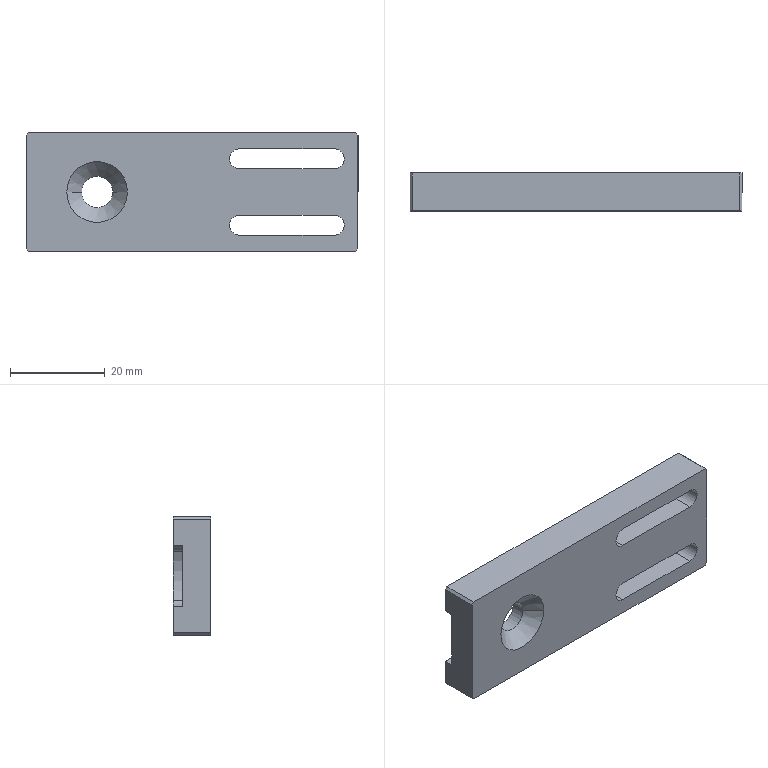Component | SolidWorks | QX1-24-TensionerSeat-1 | 1 solid | 30 faces | box 70 x 8 x 25 mm | volume 11297 mm3 | plane 17 | cylinder 11 | cone 2 | commonest cylinder face diameters 4.2 x6 6.6 x2 6 x2 19 x1 | material 6061 Alloy
build123d program:
from build123d import *

# Parameters (mm, degrees)
SKETCH1_W                                          = 70
SKETCH1_H                                          = 25
BOSS_EXTRUDE1_DEPTH                                = 8
CUT_EXTRUDE3_DEPTH                                 = 2
HOLE_SIZE_ACCORDING_TO_TYPE_1_OF_HEXAG_D           = 6.6
HOLE_SIZE_ACCORDING_TO_TYPE_1_OF_HEXAG_CSINK_D     = 12.8
HOLE_SIZE_ACCORDING_TO_TYPE_1_OF_HEXAG_CSINK_ANGLE = 90
FILLET1_R                                          = 3
CUT_EXTRUDE4_DEPTH                                 = 10
CHAMFER1_SIZE                                      = 0.5


with BuildPart() as part:
    # Sketch1 → Boss-Extrude1 (new body)
    with BuildSketch(Plane.XY):
        Rectangle(SKETCH1_W, SKETCH1_H)
    extrude(amount=BOSS_EXTRUDE1_DEPTH)

    # Sketch2 → Cut-Extrude3 (cut)
    with BuildSketch(Plane.XY.offset(8)):
        with BuildLine():
            Line((6.072, 6.5), (35, 6.5))
            Line((35, 6.5), (35, -6.5))
            Line((35, -6.5), (6.072, -6.5))
            ThreePointArc((6.072, -6.5), (3.5, 0), (6.072, 6.5))
        make_face()
    extrude(amount=-CUT_EXTRUDE3_DEPTH, mode=Mode.SUBTRACT)

    # Hole Size_ according to_ Type 1 of Hexag (through all)
    with Locations(Plane(origin=(0, 0, 0), x_dir=(-1, 0, 0), z_dir=(0, 0, -1))):
        with Locations((-20, 0)):
            CounterSinkHole(HOLE_SIZE_ACCORDING_TO_TYPE_1_OF_HEXAG_D / 2, HOLE_SIZE_ACCORDING_TO_TYPE_1_OF_HEXAG_CSINK_D / 2, counter_sink_angle=HOLE_SIZE_ACCORDING_TO_TYPE_1_OF_HEXAG_CSINK_ANGLE)

    # Fillet1
    fillet1_edges = [part.edges().sort_by_distance(p)[0] for p in [
        (6.072, -6.5, 7),
        (6.072, 6.5, 7),
    ]]
    fillet(fillet1_edges, radius=FILLET1_R)

    # Sketch7 → Cut-Extrude4 (cut)
    with BuildSketch(Plane.XY.offset(8)):
        with BuildLine():
            Line((-30, 9.1), (-10, 9.1))
            ThreePointArc((-10, 9.1), (-7.9, 7), (-10, 4.9))
            Line((-10, 4.9), (-30, 4.9))
            ThreePointArc((-30, 4.9), (-32.1, 7), (-30, 9.1))
        make_face()
    cut_extrude4 = extrude(amount=-CUT_EXTRUDE4_DEPTH, mode=Mode.SUBTRACT)

    # Mirror1: Cut-Extrude4 across plane
    add(cut_extrude4.mirror(Plane.ZX), mode=Mode.SUBTRACT)

    # Chamfer1
    chamfer1_edges = [part.edges().sort_by_distance(p)[0] for p in [
        (35, -12.5, 4),
        (-35, -12.5, 4),
        (-35, 12.5, 4),
        (35, 12.5, 4),
    ]]
    chamfer(chamfer1_edges, length=CHAMFER1_SIZE)


solid = part.part

# Placed as in the assembly
solid = solid.moved(Location((32.703, -35.916, 470.247), (-90, 0, 180)))
STEP:
#1=COLOUR_RGB('',0.7922,0.8196,0.9333);
#2=FILL_AREA_STYLE_COLOUR('',#1);
#3=FILL_AREA_STYLE('',(#2));
#4=SURFACE_STYLE_FILL_AREA(#3);
#5=SURFACE_SIDE_STYLE('',(#4));
#6=SURFACE_STYLE_USAGE(.BOTH.,#5);
#7=PRESENTATION_STYLE_ASSIGNMENT((#6));
#8=CARTESIAN_POINT('',(1.599,-1.414,18.238));
#9=VERTEX_POINT('',#8);
#10=CARTESIAN_POINT('',(1.681,-1.414,18.321));
#11=VERTEX_POINT('',#10);
#12=CARTESIAN_POINT('',(1.681,-1.414,18.238));
#13=DIRECTION('',(0.,1.,0.));
#14=DIRECTION('',(1.,0.,0.));
#15=AXIS2_PLACEMENT_3D('',#12,#13,#14);
#16=CIRCLE('',#15,0.08268);
#17=EDGE_CURVE('',#9,#11,#16,.T.);
#18=ORIENTED_EDGE('',*,*,#17,.F.);
#19=CARTESIAN_POINT('',(1.599,-1.099,18.238));
#20=VERTEX_POINT('',#19);
#21=CARTESIAN_POINT('',(1.599,-1.493,18.238));
#22=DIRECTION('',(0.,1.,0.));
#23=VECTOR('',#22,39.37);
#24=LINE('',#21,#23);
#25=EDGE_CURVE('',#9,#20,#24,.T.);
#26=ORIENTED_EDGE('',*,*,#25,.T.);
#27=CARTESIAN_POINT('',(1.681,-1.099,18.321));
#28=VERTEX_POINT('',#27);
#29=CARTESIAN_POINT('',(1.681,-1.099,18.238));
#30=DIRECTION('',(-0.,-1.,-0.));
#31=DIRECTION('',(-1.,0.,0.));
#32=AXIS2_PLACEMENT_3D('',#29,#30,#31);
#33=CIRCLE('',#32,0.08268);
#34=EDGE_CURVE('',#28,#20,#33,.T.);
#35=ORIENTED_EDGE('',*,*,#34,.F.);
#36=CARTESIAN_POINT('',(1.681,-1.493,18.321));
#37=DIRECTION('',(0.,1.,0.));
#38=VECTOR('',#37,39.37);
#39=LINE('',#36,#38);
#40=EDGE_CURVE('',#11,#28,#39,.T.);
#41=ORIENTED_EDGE('',*,*,#40,.F.);
#42=EDGE_LOOP('',(#18,#26,#35,#41));
#43=FACE_OUTER_BOUND('',#42,.T.);
#44=CARTESIAN_POINT('',(1.681,-1.493,18.238));
#45=DIRECTION('',(0.,1.,0.));
#46=DIRECTION('',(-1.,0.,0.));
#47=AXIS2_PLACEMENT_3D('',#44,#45,#46);
#48=CYLINDRICAL_SURFACE('',#47,0.08268);
#49=ADVANCED_FACE('',(#43),#48,.F.);
#50=CARTESIAN_POINT('',(1.681,-1.414,18.872));
#51=VERTEX_POINT('',#50);
#52=CARTESIAN_POINT('',(1.599,-1.414,18.789));
#53=VERTEX_POINT('',#52);
#54=CARTESIAN_POINT('',(1.681,-1.414,18.789));
#55=DIRECTION('',(-0.,-1.,-0.));
#56=DIRECTION('',(1.,0.,0.));
#57=AXIS2_PLACEMENT_3D('',#54,#55,#56);
#58=CIRCLE('',#57,0.08268);
#59=EDGE_CURVE('',#51,#53,#58,.T.);
#60=ORIENTED_EDGE('',*,*,#59,.T.);
#61=CARTESIAN_POINT('',(1.599,-1.099,18.789));
#62=VERTEX_POINT('',#61);
#63=CARTESIAN_POINT('',(1.599,-1.493,18.789));
#64=DIRECTION('',(0.,1.,0.));
#65=VECTOR('',#64,39.37);
#66=LINE('',#63,#65);
#67=EDGE_CURVE('',#53,#62,#66,.T.);
#68=ORIENTED_EDGE('',*,*,#67,.T.);
#69=CARTESIAN_POINT('',(1.681,-1.099,18.872));
#70=VERTEX_POINT('',#69);
#71=CARTESIAN_POINT('',(1.681,-1.099,18.789));
#72=DIRECTION('',(0.,1.,0.));
#73=DIRECTION('',(-1.,0.,0.));
#74=AXIS2_PLACEMENT_3D('',#71,#72,#73);
#75=CIRCLE('',#74,0.08268);
#76=EDGE_CURVE('',#62,#70,#75,.T.);
#77=ORIENTED_EDGE('',*,*,#76,.T.);
#78=CARTESIAN_POINT('',(1.681,-1.493,18.872));
#79=DIRECTION('',(0.,1.,0.));
#80=VECTOR('',#79,39.37);
#81=LINE('',#78,#80);
#82=EDGE_CURVE('',#51,#70,#81,.T.);
#83=ORIENTED_EDGE('',*,*,#82,.F.);
#84=EDGE_LOOP('',(#60,#68,#77,#83));
#85=FACE_OUTER_BOUND('',#84,.T.);
#86=CARTESIAN_POINT('',(1.681,-1.493,18.789));
#87=DIRECTION('',(0.,1.,0.));
#88=DIRECTION('',(-1.,0.,0.));
#89=AXIS2_PLACEMENT_3D('',#86,#87,#88);
#90=CYLINDRICAL_SURFACE('',#89,0.08268);
#91=ADVANCED_FACE('',(#85),#90,.F.);
#92=CARTESIAN_POINT('',(0.3702,-1.292,18.514));
#93=VERTEX_POINT('',#92);
#94=CARTESIAN_POINT('',(0.6301,-1.292,18.514));
#95=VERTEX_POINT('',#94);
#96=CARTESIAN_POINT('',(0.5001,-1.292,18.514));
#97=DIRECTION('',(-0.,-1.,-0.));
#98=DIRECTION('',(1.,0.,0.));
#99=AXIS2_PLACEMENT_3D('',#96,#97,#98);
#100=CIRCLE('',#99,0.1299);
#101=EDGE_CURVE('',#93,#95,#100,.T.);
#102=ORIENTED_EDGE('',*,*,#101,.F.);
#103=CARTESIAN_POINT('',(0.2482,-1.414,18.514));
#104=VERTEX_POINT('',#103);
#105=CARTESIAN_POINT('',(0.2482,-1.414,18.514));
#106=DIRECTION('',(-0.7071,-0.7071,0.));
#107=VECTOR('',#106,39.37);
#108=LINE('',#105,#107);
#109=EDGE_CURVE('',#93,#104,#108,.T.);
#110=ORIENTED_EDGE('',*,*,#109,.T.);
#111=CARTESIAN_POINT('',(0.7521,-1.414,18.514));
#112=VERTEX_POINT('',#111);
#113=CARTESIAN_POINT('',(0.5001,-1.414,18.514));
#114=DIRECTION('',(-0.,-1.,-0.));
#115=DIRECTION('',(1.,-0.,0.));
#116=AXIS2_PLACEMENT_3D('',#113,#114,#115);
#117=CIRCLE('',#116,0.252);
#118=EDGE_CURVE('',#104,#112,#117,.T.);
#119=ORIENTED_EDGE('',*,*,#118,.T.);
#120=CARTESIAN_POINT('',(0.7521,-1.414,18.514));
#121=DIRECTION('',(0.7071,-0.7071,-0.));
#122=VECTOR('',#121,39.37);
#123=LINE('',#120,#122);
#124=EDGE_CURVE('',#95,#112,#123,.T.);
#125=ORIENTED_EDGE('',*,*,#124,.F.);
#126=EDGE_LOOP('',(#102,#110,#119,#125));
#127=FACE_OUTER_BOUND('',#126,.T.);
#128=CARTESIAN_POINT('',(0.5001,-1.414,18.514));
#129=DIRECTION('',(-0.,-1.,-0.));
#130=DIRECTION('',(1.,-0.,0.));
#131=AXIS2_PLACEMENT_3D('',#128,#129,#130);
#132=CONICAL_SURFACE('',#131,0.252,0.7854);
#133=ADVANCED_FACE('',(#127),#132,.F.);
#134=CARTESIAN_POINT('',(0.6301,-1.178,18.514));
#135=VERTEX_POINT('',#134);
#136=CARTESIAN_POINT('',(0.3702,-1.178,18.514));
#137=VERTEX_POINT('',#136);
#138=CARTESIAN_POINT('',(0.5001,-1.178,18.514));
#139=DIRECTION('',(0.,1.,0.));
#140=DIRECTION('',(-1.,0.,0.));
#141=AXIS2_PLACEMENT_3D('',#138,#139,#140);
#142=CIRCLE('',#141,0.1299);
#143=EDGE_CURVE('',#135,#137,#142,.T.);
#144=ORIENTED_EDGE('',*,*,#143,.T.);
#145=CARTESIAN_POINT('',(0.3702,-1.414,18.514));
#146=DIRECTION('',(-0.,-1.,-0.));
#147=VECTOR('',#146,39.37);
#148=LINE('',#145,#147);
#149=EDGE_CURVE('',#137,#93,#148,.T.);
#150=ORIENTED_EDGE('',*,*,#149,.T.);
#151=ORIENTED_EDGE('',*,*,#101,.T.);
#152=CARTESIAN_POINT('',(0.6301,-1.414,18.514));
#153=DIRECTION('',(-0.,-1.,-0.));
#154=VECTOR('',#153,39.37);
#155=LINE('',#152,#154);
#156=EDGE_CURVE('',#135,#95,#155,.T.);
#157=ORIENTED_EDGE('',*,*,#156,.F.);
#158=EDGE_LOOP('',(#144,#150,#151,#157));
#159=FACE_OUTER_BOUND('',#158,.T.);
#160=CARTESIAN_POINT('',(0.5001,-1.414,18.514));
#161=DIRECTION('',(-0.,-1.,-0.));
#162=DIRECTION('',(1.,0.,0.));
#163=AXIS2_PLACEMENT_3D('',#160,#161,#162);
#164=CYLINDRICAL_SURFACE('',#163,0.1299);
#165=ADVANCED_FACE('',(#159),#164,.F.);
#166=CARTESIAN_POINT('',(-0.09042,-1.099,18.77));
#167=VERTEX_POINT('',#166);
#168=CARTESIAN_POINT('',(-0.09042,-1.099,18.986));
#169=VERTEX_POINT('',#168);
#170=CARTESIAN_POINT('',(-0.09042,-1.099,18.022));
#171=DIRECTION('',(0.,-0.,1.));
#172=VECTOR('',#171,39.37);
#173=LINE('',#170,#172);
#174=EDGE_CURVE('',#167,#169,#173,.T.);
#175=ORIENTED_EDGE('',*,*,#174,.T.);
#176=CARTESIAN_POINT('',(-0.07074,-1.099,19.006));
#177=VERTEX_POINT('',#176);
#178=CARTESIAN_POINT('',(-0.07074,-1.099,19.006));
#179=DIRECTION('',(0.7071,-0.,0.7071));
#180=VECTOR('',#179,39.37);
#181=LINE('',#178,#180);
#182=EDGE_CURVE('',#169,#177,#181,.T.);
#183=ORIENTED_EDGE('',*,*,#182,.T.);
#184=CARTESIAN_POINT('',(2.646,-1.099,19.006));
#185=VERTEX_POINT('',#184);
#186=CARTESIAN_POINT('',(2.665,-1.099,19.006));
#187=DIRECTION('',(1.,-0.,-0.));
#188=VECTOR('',#187,39.37);
#189=LINE('',#186,#188);
#190=EDGE_CURVE('',#177,#185,#189,.T.);
#191=ORIENTED_EDGE('',*,*,#190,.T.);
#192=CARTESIAN_POINT('',(2.665,-1.099,18.986));
#193=VERTEX_POINT('',#192);
#194=CARTESIAN_POINT('',(2.665,-1.099,18.986));
#195=DIRECTION('',(0.7071,-0.,-0.7071));
#196=VECTOR('',#195,39.37);
#197=LINE('',#194,#196);
#198=EDGE_CURVE('',#185,#193,#197,.T.);
#199=ORIENTED_EDGE('',*,*,#198,.T.);
#200=CARTESIAN_POINT('',(2.665,-1.099,18.041));
#201=VERTEX_POINT('',#200);
#202=CARTESIAN_POINT('',(2.665,-1.099,18.022));
#203=DIRECTION('',(-0.,0.,-1.));
#204=VECTOR('',#203,39.37);
#205=LINE('',#202,#204);
#206=EDGE_CURVE('',#193,#201,#205,.T.);
#207=ORIENTED_EDGE('',*,*,#206,.T.);
#208=CARTESIAN_POINT('',(2.646,-1.099,18.022));
#209=VERTEX_POINT('',#208);
#210=CARTESIAN_POINT('',(2.646,-1.099,18.022));
#211=DIRECTION('',(-0.7071,0.,-0.7071));
#212=VECTOR('',#211,39.37);
#213=LINE('',#210,#212);
#214=EDGE_CURVE('',#201,#209,#213,.T.);
#215=ORIENTED_EDGE('',*,*,#214,.T.);
#216=CARTESIAN_POINT('',(-0.07074,-1.099,18.022));
#217=VERTEX_POINT('',#216);
#218=CARTESIAN_POINT('',(2.665,-1.099,18.022));
#219=DIRECTION('',(-1.,0.,0.));
#220=VECTOR('',#219,39.37);
#221=LINE('',#218,#220);
#222=EDGE_CURVE('',#209,#217,#221,.T.);
#223=ORIENTED_EDGE('',*,*,#222,.T.);
#224=CARTESIAN_POINT('',(-0.09042,-1.099,18.041));
#225=VERTEX_POINT('',#224);
#226=CARTESIAN_POINT('',(-0.09042,-1.099,18.041));
#227=DIRECTION('',(-0.7071,0.,0.7071));
#228=VECTOR('',#227,39.37);
#229=LINE('',#226,#228);
#230=EDGE_CURVE('',#217,#225,#229,.T.);
#231=ORIENTED_EDGE('',*,*,#230,.T.);
#232=CARTESIAN_POINT('',(-0.09042,-1.099,18.258));
#233=VERTEX_POINT('',#232);
#234=CARTESIAN_POINT('',(-0.09042,-1.099,18.022));
#235=DIRECTION('',(0.,-0.,1.));
#236=VECTOR('',#235,39.37);
#237=LINE('',#234,#236);
#238=EDGE_CURVE('',#225,#233,#237,.T.);
#239=ORIENTED_EDGE('',*,*,#238,.T.);
#240=CARTESIAN_POINT('',(0.9914,-1.099,18.258));
#241=VERTEX_POINT('',#240);
#242=CARTESIAN_POINT('',(1.048,-1.099,18.258));
#243=DIRECTION('',(-1.,0.,0.));
#244=VECTOR('',#243,39.37);
#245=LINE('',#242,#244);
#246=EDGE_CURVE('',#241,#233,#245,.T.);
#247=ORIENTED_EDGE('',*,*,#246,.F.);
#248=CARTESIAN_POINT('',(1.091,-1.099,18.312));
#249=VERTEX_POINT('',#248);
#250=CARTESIAN_POINT('',(0.9914,-1.099,18.376));
#251=DIRECTION('',(-0.,-1.,-0.));
#252=DIRECTION('',(1.,-0.,0.));
#253=AXIS2_PLACEMENT_3D('',#250,#251,#252);
#254=CIRCLE('',#253,0.1181);
#255=EDGE_CURVE('',#241,#249,#254,.T.);
#256=ORIENTED_EDGE('',*,*,#255,.T.);
#257=CARTESIAN_POINT('',(1.091,-1.099,18.715));
#258=VERTEX_POINT('',#257);
#259=CARTESIAN_POINT('',(0.7757,-1.099,18.514));
#260=DIRECTION('',(0.,1.,0.));
#261=DIRECTION('',(-1.,0.,0.));
#262=AXIS2_PLACEMENT_3D('',#259,#260,#261);
#263=CIRCLE('',#262,0.374);
#264=EDGE_CURVE('',#258,#249,#263,.T.);
#265=ORIENTED_EDGE('',*,*,#264,.F.);
#266=CARTESIAN_POINT('',(0.9914,-1.099,18.77));
#267=VERTEX_POINT('',#266);
#268=CARTESIAN_POINT('',(0.9914,-1.099,18.651));
#269=DIRECTION('',(-0.,-1.,-0.));
#270=DIRECTION('',(1.,-0.,0.));
#271=AXIS2_PLACEMENT_3D('',#268,#269,#270);
#272=CIRCLE('',#271,0.1181);
#273=EDGE_CURVE('',#258,#267,#272,.T.);
#274=ORIENTED_EDGE('',*,*,#273,.T.);
#275=CARTESIAN_POINT('',(1.048,-1.099,18.77));
#276=DIRECTION('',(-1.,0.,0.));
#277=VECTOR('',#276,39.37);
#278=LINE('',#275,#277);
#279=EDGE_CURVE('',#267,#167,#278,.T.);
#280=ORIENTED_EDGE('',*,*,#279,.T.);
#281=EDGE_LOOP('',(#175,#183,#191,#199,#207,#215,#223,#231,#239,#247,#256,#265,#274,#280));
#282=FACE_OUTER_BOUND('',#281,.T.);
#283=CARTESIAN_POINT('',(2.469,-1.099,18.707));
#284=VERTEX_POINT('',#283);
#285=CARTESIAN_POINT('',(1.681,-1.099,18.707));
#286=VERTEX_POINT('',#285);
#287=CARTESIAN_POINT('',(2.469,-1.099,18.707));
#288=DIRECTION('',(-1.,0.,0.));
#289=VECTOR('',#288,39.37);
#290=LINE('',#287,#289);
#291=EDGE_CURVE('',#284,#286,#290,.T.);
#292=ORIENTED_EDGE('',*,*,#291,.F.);
#293=CARTESIAN_POINT('',(2.469,-1.099,18.872));
#294=VERTEX_POINT('',#293);
#295=CARTESIAN_POINT('',(2.469,-1.099,18.789));
#296=DIRECTION('',(0.,1.,0.));
#297=DIRECTION('',(-1.,0.,0.));
#298=AXIS2_PLACEMENT_3D('',#295,#296,#297);
#299=CIRCLE('',#298,0.08268);
#300=EDGE_CURVE('',#294,#284,#299,.T.);
#301=ORIENTED_EDGE('',*,*,#300,.F.);
#302=CARTESIAN_POINT('',(2.469,-1.099,18.872));
#303=DIRECTION('',(1.,-0.,-0.));
#304=VECTOR('',#303,39.37);
#305=LINE('',#302,#304);
#306=EDGE_CURVE('',#70,#294,#305,.T.);
#307=ORIENTED_EDGE('',*,*,#306,.F.);
#308=ORIENTED_EDGE('',*,*,#76,.F.);
#309=CARTESIAN_POINT('',(1.681,-1.099,18.789));
#310=DIRECTION('',(0.,1.,0.));
#311=DIRECTION('',(-1.,0.,0.));
#312=AXIS2_PLACEMENT_3D('',#309,#310,#311);
#313=CIRCLE('',#312,0.08268);
#314=EDGE_CURVE('',#286,#62,#313,.T.);
#315=ORIENTED_EDGE('',*,*,#314,.F.);
#316=EDGE_LOOP('',(#292,#301,#307,#308,#315));
#317=FACE_BOUND('',#316,.T.);
#318=CARTESIAN_POINT('',(2.469,-1.099,18.155));
#319=VERTEX_POINT('',#318);
#320=CARTESIAN_POINT('',(2.469,-1.099,18.321));
#321=VERTEX_POINT('',#320);
#322=CARTESIAN_POINT('',(2.469,-1.099,18.238));
#323=DIRECTION('',(-0.,-1.,-0.));
#324=DIRECTION('',(-1.,0.,0.));
#325=AXIS2_PLACEMENT_3D('',#322,#323,#324);
#326=CIRCLE('',#325,0.08268);
#327=EDGE_CURVE('',#319,#321,#326,.T.);
#328=ORIENTED_EDGE('',*,*,#327,.T.);
#329=CARTESIAN_POINT('',(2.469,-1.099,18.321));
#330=DIRECTION('',(-1.,0.,0.));
#331=VECTOR('',#330,39.37);
#332=LINE('',#329,#331);
#333=EDGE_CURVE('',#321,#28,#332,.T.);
#334=ORIENTED_EDGE('',*,*,#333,.T.);
#335=ORIENTED_EDGE('',*,*,#34,.T.);
#336=CARTESIAN_POINT('',(1.681,-1.099,18.155));
#337=VERTEX_POINT('',#336);
#338=CARTESIAN_POINT('',(1.681,-1.099,18.238));
#339=DIRECTION('',(-0.,-1.,-0.));
#340=DIRECTION('',(-1.,0.,0.));
#341=AXIS2_PLACEMENT_3D('',#338,#339,#340);
#342=CIRCLE('',#341,0.08268);
#343=EDGE_CURVE('',#20,#337,#342,.T.);
#344=ORIENTED_EDGE('',*,*,#343,.T.);
#345=CARTESIAN_POINT('',(2.469,-1.099,18.155));
#346=DIRECTION('',(1.,-0.,-0.));
#347=VECTOR('',#346,39.37);
#348=LINE('',#345,#347);
#349=EDGE_CURVE('',#337,#319,#348,.T.);
#350=ORIENTED_EDGE('',*,*,#349,.T.);
#351=EDGE_LOOP('',(#328,#334,#335,#344,#350));
#352=FACE_BOUND('',#351,.T.);
#353=CARTESIAN_POINT('',(1.288,-1.099,18.514));
#354=DIRECTION('',(-0.,-1.,-0.));
#355=DIRECTION('',(1.,-0.,-0.));
#356=AXIS2_PLACEMENT_3D('',#353,#354,#355);
#357=PLANE('',#356);
#358=ADVANCED_FACE('',(#282,#317,#352),#357,.F.);
#359=CARTESIAN_POINT('',(2.469,-1.414,18.707));
#360=VERTEX_POINT('',#359);
#361=CARTESIAN_POINT('',(2.469,-1.414,18.872));
#362=VERTEX_POINT('',#361);
#363=CARTESIAN_POINT('',(2.469,-1.414,18.789));
#364=DIRECTION('',(-0.,-1.,-0.));
#365=DIRECTION('',(1.,0.,0.));
#366=AXIS2_PLACEMENT_3D('',#363,#364,#365);
#367=CIRCLE('',#366,0.08268);
#368=EDGE_CURVE('',#360,#362,#367,.T.);
#369=ORIENTED_EDGE('',*,*,#368,.F.);
#370=CARTESIAN_POINT('',(1.681,-1.414,18.707));
#371=VERTEX_POINT('',#370);
#372=CARTESIAN_POINT('',(1.288,-1.414,18.707));
#373=DIRECTION('',(1.,-0.,-0.));
#374=VECTOR('',#373,39.37);
#375=LINE('',#372,#374);
#376=EDGE_CURVE('',#371,#360,#375,.T.);
#377=ORIENTED_EDGE('',*,*,#376,.F.);
#378=CARTESIAN_POINT('',(1.681,-1.414,18.789));
#379=DIRECTION('',(-0.,-1.,-0.));
#380=DIRECTION('',(1.,0.,0.));
#381=AXIS2_PLACEMENT_3D('',#378,#379,#380);
#382=CIRCLE('',#381,0.08268);
#383=EDGE_CURVE('',#53,#371,#382,.T.);
#384=ORIENTED_EDGE('',*,*,#383,.F.);
#385=ORIENTED_EDGE('',*,*,#59,.F.);
#386=CARTESIAN_POINT('',(1.288,-1.414,18.872));
#387=DIRECTION('',(-1.,0.,0.));
#388=VECTOR('',#387,39.37);
#389=LINE('',#386,#388);
#390=EDGE_CURVE('',#362,#51,#389,.T.);
#391=ORIENTED_EDGE('',*,*,#390,.F.);
#392=EDGE_LOOP('',(#369,#377,#384,#385,#391));
#393=FACE_BOUND('',#392,.T.);
#394=CARTESIAN_POINT('',(0.5001,-1.414,18.514));
#395=DIRECTION('',(-0.,-1.,-0.));
#396=DIRECTION('',(1.,-0.,0.));
#397=AXIS2_PLACEMENT_3D('',#394,#395,#396);
#398=CIRCLE('',#397,0.252);
#399=EDGE_CURVE('',#112,#104,#398,.T.);
#400=ORIENTED_EDGE('',*,*,#399,.F.);
#401=ORIENTED_EDGE('',*,*,#118,.F.);
#402=EDGE_LOOP('',(#400,#401));
#403=FACE_BOUND('',#402,.T.);
#404=CARTESIAN_POINT('',(-0.07074,-1.414,19.006));
#405=VERTEX_POINT('',#404);
#406=CARTESIAN_POINT('',(2.646,-1.414,19.006));
#407=VERTEX_POINT('',#406);
#408=CARTESIAN_POINT('',(2.665,-1.414,19.006));
#409=DIRECTION('',(1.,-0.,-0.));
#410=VECTOR('',#409,39.37);
#411=LINE('',#408,#410);
#412=EDGE_CURVE('',#405,#407,#411,.T.);
#413=ORIENTED_EDGE('',*,*,#412,.F.);
#414=CARTESIAN_POINT('',(-0.09042,-1.414,18.986));
#415=VERTEX_POINT('',#414);
#416=CARTESIAN_POINT('',(0.3623,-1.414,19.439));
#417=DIRECTION('',(-0.7071,0.,-0.7071));
#418=VECTOR('',#417,39.37);
#419=LINE('',#416,#418);
#420=EDGE_CURVE('',#405,#415,#419,.T.);
#421=ORIENTED_EDGE('',*,*,#420,.T.);
#422=CARTESIAN_POINT('',(-0.09042,-1.414,18.041));
#423=VERTEX_POINT('',#422);
#424=CARTESIAN_POINT('',(-0.09042,-1.414,18.022));
#425=DIRECTION('',(0.,-0.,1.));
#426=VECTOR('',#425,39.37);
#427=LINE('',#424,#426);
#428=EDGE_CURVE('',#423,#415,#427,.T.);
#429=ORIENTED_EDGE('',*,*,#428,.F.);
#430=CARTESIAN_POINT('',(-0.07074,-1.414,18.022));
#431=VERTEX_POINT('',#430);
#432=CARTESIAN_POINT('',(0.3623,-1.414,17.588));
#433=DIRECTION('',(0.7071,-0.,-0.7071));
#434=VECTOR('',#433,39.37);
#435=LINE('',#432,#434);
#436=EDGE_CURVE('',#423,#431,#435,.T.);
#437=ORIENTED_EDGE('',*,*,#436,.T.);
#438=CARTESIAN_POINT('',(2.646,-1.414,18.022));
#439=VERTEX_POINT('',#438);
#440=CARTESIAN_POINT('',(2.665,-1.414,18.022));
#441=DIRECTION('',(-1.,0.,0.));
#442=VECTOR('',#441,39.37);
#443=LINE('',#440,#442);
#444=EDGE_CURVE('',#439,#431,#443,.T.);
#445=ORIENTED_EDGE('',*,*,#444,.F.);
#446=CARTESIAN_POINT('',(2.665,-1.414,18.041));
#447=VERTEX_POINT('',#446);
#448=CARTESIAN_POINT('',(2.213,-1.414,17.588));
#449=DIRECTION('',(0.7071,-0.,0.7071));
#450=VECTOR('',#449,39.37);
#451=LINE('',#448,#450);
#452=EDGE_CURVE('',#439,#447,#451,.T.);
#453=ORIENTED_EDGE('',*,*,#452,.T.);
#454=CARTESIAN_POINT('',(2.665,-1.414,18.986));
#455=VERTEX_POINT('',#454);
#456=CARTESIAN_POINT('',(2.665,-1.414,18.022));
#457=DIRECTION('',(-0.,0.,-1.));
#458=VECTOR('',#457,39.37);
#459=LINE('',#456,#458);
#460=EDGE_CURVE('',#455,#447,#459,.T.);
#461=ORIENTED_EDGE('',*,*,#460,.F.);
#462=CARTESIAN_POINT('',(2.213,-1.414,19.439));
#463=DIRECTION('',(-0.7071,0.,0.7071));
#464=VECTOR('',#463,39.37);
#465=LINE('',#462,#464);
#466=EDGE_CURVE('',#455,#407,#465,.T.);
#467=ORIENTED_EDGE('',*,*,#466,.T.);
#468=EDGE_LOOP('',(#413,#421,#429,#437,#445,#453,#461,#467));
#469=FACE_OUTER_BOUND('',#468,.T.);
#470=CARTESIAN_POINT('',(2.469,-1.414,18.321));
#471=VERTEX_POINT('',#470);
#472=CARTESIAN_POINT('',(1.288,-1.414,18.321));
#473=DIRECTION('',(1.,-0.,-0.));
#474=VECTOR('',#473,39.37);
#475=LINE('',#472,#474);
#476=EDGE_CURVE('',#11,#471,#475,.T.);
#477=ORIENTED_EDGE('',*,*,#476,.T.);
#478=CARTESIAN_POINT('',(2.469,-1.414,18.155));
#479=VERTEX_POINT('',#478);
#480=CARTESIAN_POINT('',(2.469,-1.414,18.238));
#481=DIRECTION('',(0.,1.,0.));
#482=DIRECTION('',(1.,0.,0.));
#483=AXIS2_PLACEMENT_3D('',#480,#481,#482);
#484=CIRCLE('',#483,0.08268);
#485=EDGE_CURVE('',#471,#479,#484,.T.);
#486=ORIENTED_EDGE('',*,*,#485,.T.);
#487=CARTESIAN_POINT('',(1.681,-1.414,18.155));
#488=VERTEX_POINT('',#487);
#489=CARTESIAN_POINT('',(1.288,-1.414,18.155));
#490=DIRECTION('',(-1.,0.,0.));
#491=VECTOR('',#490,39.37);
#492=LINE('',#489,#491);
#493=EDGE_CURVE('',#479,#488,#492,.T.);
#494=ORIENTED_EDGE('',*,*,#493,.T.);
#495=CARTESIAN_POINT('',(1.681,-1.414,18.238));
#496=DIRECTION('',(0.,1.,0.));
#497=DIRECTION('',(1.,0.,0.));
#498=AXIS2_PLACEMENT_3D('',#495,#496,#497);
#499=CIRCLE('',#498,0.08268);
#500=EDGE_CURVE('',#488,#9,#499,.T.);
#501=ORIENTED_EDGE('',*,*,#500,.T.);
#502=ORIENTED_EDGE('',*,*,#17,.T.);
#503=EDGE_LOOP('',(#477,#486,#494,#501,#502));
#504=FACE_BOUND('',#503,.T.);
#505=CARTESIAN_POINT('',(1.288,-1.414,18.514));
#506=DIRECTION('',(-0.,-1.,-0.));
#507=DIRECTION('',(1.,-0.,-0.));
#508=AXIS2_PLACEMENT_3D('',#505,#506,#507);
#509=PLANE('',#508);
#510=ADVANCED_FACE('',(#393,#403,#469,#504),#509,.T.);
#511=ORIENTED_EDGE('',*,*,#428,.T.);
#512=CARTESIAN_POINT('',(-0.09042,-1.099,18.986));
#513=DIRECTION('',(0.,1.,0.));
#514=VECTOR('',#513,39.37);
#515=LINE('',#512,#514);
#516=EDGE_CURVE('',#415,#169,#515,.T.);
#517=ORIENTED_EDGE('',*,*,#516,.T.);
#518=ORIENTED_EDGE('',*,*,#174,.F.);
#519=CARTESIAN_POINT('',(-0.09042,-1.178,18.77));
#520=VERTEX_POINT('',#519);
#521=CARTESIAN_POINT('',(-0.09042,-1.178,18.77));
#522=DIRECTION('',(0.,1.,0.));
#523=VECTOR('',#522,39.37);
#524=LINE('',#521,#523);
#525=EDGE_CURVE('',#520,#167,#524,.T.);
#526=ORIENTED_EDGE('',*,*,#525,.F.);
#527=CARTESIAN_POINT('',(-0.09042,-1.178,18.258));
#528=VERTEX_POINT('',#527);
#529=CARTESIAN_POINT('',(-0.09042,-1.178,18.77));
#530=DIRECTION('',(-0.,0.,-1.));
#531=VECTOR('',#530,39.37);
#532=LINE('',#529,#531);
#533=EDGE_CURVE('',#520,#528,#532,.T.);
#534=ORIENTED_EDGE('',*,*,#533,.T.);
#535=CARTESIAN_POINT('',(-0.09042,-1.178,18.258));
#536=DIRECTION('',(0.,1.,0.));
#537=VECTOR('',#536,39.37);
#538=LINE('',#535,#537);
#539=EDGE_CURVE('',#528,#233,#538,.T.);
#540=ORIENTED_EDGE('',*,*,#539,.T.);
#541=ORIENTED_EDGE('',*,*,#238,.F.);
#542=CARTESIAN_POINT('',(-0.09042,-1.099,18.041));
#543=DIRECTION('',(-0.,-1.,-0.));
#544=VECTOR('',#543,39.37);
#545=LINE('',#542,#544);
#546=EDGE_CURVE('',#225,#423,#545,.T.);
#547=ORIENTED_EDGE('',*,*,#546,.T.);
#548=EDGE_LOOP('',(#511,#517,#518,#526,#534,#540,#541,#547));
#549=FACE_OUTER_BOUND('',#548,.T.);
#550=CARTESIAN_POINT('',(-0.09042,-1.099,18.022));
#551=DIRECTION('',(1.,-0.,-0.));
#552=DIRECTION('',(0.,1.,0.));
#553=AXIS2_PLACEMENT_3D('',#550,#551,#552);
#554=PLANE('',#553);
#555=ADVANCED_FACE('',(#549),#554,.F.);
#556=ORIENTED_EDGE('',*,*,#190,.F.);
#557=CARTESIAN_POINT('',(-0.07074,-1.099,19.006));
#558=DIRECTION('',(-0.,-1.,-0.));
#559=VECTOR('',#558,39.37);
#560=LINE('',#557,#559);
#561=EDGE_CURVE('',#177,#405,#560,.T.);
#562=ORIENTED_EDGE('',*,*,#561,.T.);
#563=ORIENTED_EDGE('',*,*,#412,.T.);
#564=CARTESIAN_POINT('',(2.646,-1.099,19.006));
#565=DIRECTION('',(0.,1.,0.));
#566=VECTOR('',#565,39.37);
#567=LINE('',#564,#566);
#568=EDGE_CURVE('',#407,#185,#567,.T.);
#569=ORIENTED_EDGE('',*,*,#568,.T.);
#570=EDGE_LOOP('',(#556,#562,#563,#569));
#571=FACE_OUTER_BOUND('',#570,.T.);
#572=CARTESIAN_POINT('',(2.665,-1.099,19.006));
#573=DIRECTION('',(-0.,0.,-1.));
#574=DIRECTION('',(-0.,-1.,-0.));
#575=AXIS2_PLACEMENT_3D('',#572,#573,#574);
#576=PLANE('',#575);
#577=ADVANCED_FACE('',(#571),#576,.F.);
#578=ORIENTED_EDGE('',*,*,#460,.T.);
#579=CARTESIAN_POINT('',(2.665,-1.099,18.041));
#580=DIRECTION('',(0.,1.,0.));
#581=VECTOR('',#580,39.37);
#582=LINE('',#579,#581);
#583=EDGE_CURVE('',#447,#201,#582,.T.);
#584=ORIENTED_EDGE('',*,*,#583,.T.);
#585=ORIENTED_EDGE('',*,*,#206,.F.);
#586=CARTESIAN_POINT('',(2.665,-1.099,18.986));
#587=DIRECTION('',(-0.,-1.,-0.));
#588=VECTOR('',#587,39.37);
#589=LINE('',#586,#588);
#590=EDGE_CURVE('',#193,#455,#589,.T.);
#591=ORIENTED_EDGE('',*,*,#590,.T.);
#592=EDGE_LOOP('',(#578,#584,#585,#591));
#593=FACE_OUTER_BOUND('',#592,.T.);
#594=CARTESIAN_POINT('',(2.665,-1.099,18.022));
#595=DIRECTION('',(-1.,0.,0.));
#596=DIRECTION('',(-0.,-1.,-0.));
#597=AXIS2_PLACEMENT_3D('',#594,#595,#596);
#598=PLANE('',#597);
#599=ADVANCED_FACE('',(#593),#598,.F.);
#600=ORIENTED_EDGE('',*,*,#444,.T.);
#601=CARTESIAN_POINT('',(-0.07074,-1.099,18.022));
#602=DIRECTION('',(0.,1.,0.));
#603=VECTOR('',#602,39.37);
#604=LINE('',#601,#603);
#605=EDGE_CURVE('',#431,#217,#604,.T.);
#606=ORIENTED_EDGE('',*,*,#605,.T.);
#607=ORIENTED_EDGE('',*,*,#222,.F.);
#608=CARTESIAN_POINT('',(2.646,-1.099,18.022));
#609=DIRECTION('',(-0.,-1.,-0.));
#610=VECTOR('',#609,39.37);
#611=LINE('',#608,#610);
#612=EDGE_CURVE('',#209,#439,#611,.T.);
#613=ORIENTED_EDGE('',*,*,#612,.T.);
#614=EDGE_LOOP('',(#600,#606,#607,#613));
#615=FACE_OUTER_BOUND('',#614,.T.);
#616=CARTESIAN_POINT('',(2.665,-1.099,18.022));
#617=DIRECTION('',(0.,-0.,1.));
#618=DIRECTION('',(0.,1.,0.));
#619=AXIS2_PLACEMENT_3D('',#616,#617,#618);
#620=PLANE('',#619);
#621=ADVANCED_FACE('',(#615),#620,.F.);
#622=ORIENTED_EDGE('',*,*,#264,.T.);
#623=CARTESIAN_POINT('',(1.091,-1.178,18.312));
#624=VERTEX_POINT('',#623);
#625=CARTESIAN_POINT('',(1.091,-1.178,18.312));
#626=DIRECTION('',(-0.,-1.,-0.));
#627=VECTOR('',#626,39.37);
#628=LINE('',#625,#627);
#629=EDGE_CURVE('',#249,#624,#628,.T.);
#630=ORIENTED_EDGE('',*,*,#629,.T.);
#631=CARTESIAN_POINT('',(1.091,-1.178,18.715));
#632=VERTEX_POINT('',#631);
#633=CARTESIAN_POINT('',(0.7757,-1.178,18.514));
#634=DIRECTION('',(0.,1.,0.));
#635=DIRECTION('',(-1.,0.,0.));
#636=AXIS2_PLACEMENT_3D('',#633,#634,#635);
#637=CIRCLE('',#636,0.374);
#638=EDGE_CURVE('',#632,#624,#637,.T.);
#639=ORIENTED_EDGE('',*,*,#638,.F.);
#640=CARTESIAN_POINT('',(1.091,-1.178,18.715));
#641=DIRECTION('',(0.,1.,0.));
#642=VECTOR('',#641,39.37);
#643=LINE('',#640,#642);
#644=EDGE_CURVE('',#632,#258,#643,.T.);
#645=ORIENTED_EDGE('',*,*,#644,.T.);
#646=EDGE_LOOP('',(#622,#630,#639,#645));
#647=FACE_OUTER_BOUND('',#646,.T.);
#648=CARTESIAN_POINT('',(0.7757,-1.178,18.514));
#649=DIRECTION('',(0.,1.,0.));
#650=DIRECTION('',(-1.,0.,0.));
#651=AXIS2_PLACEMENT_3D('',#648,#649,#650);
#652=CYLINDRICAL_SURFACE('',#651,0.374);
#653=ADVANCED_FACE('',(#647),#652,.F.);
#654=ORIENTED_EDGE('',*,*,#279,.F.);
#655=CARTESIAN_POINT('',(0.9914,-1.178,18.77));
#656=VERTEX_POINT('',#655);
#657=CARTESIAN_POINT('',(0.9914,-1.178,18.77));
#658=DIRECTION('',(-0.,-1.,-0.));
#659=VECTOR('',#658,39.37);
#660=LINE('',#657,#659);
#661=EDGE_CURVE('',#267,#656,#660,.T.);
#662=ORIENTED_EDGE('',*,*,#661,.T.);
#663=CARTESIAN_POINT('',(1.048,-1.178,18.77));
#664=DIRECTION('',(-1.,0.,0.));
#665=VECTOR('',#664,39.37);
#666=LINE('',#663,#665);
#667=EDGE_CURVE('',#656,#520,#666,.T.);
#668=ORIENTED_EDGE('',*,*,#667,.T.);
#669=ORIENTED_EDGE('',*,*,#525,.T.);
#670=EDGE_LOOP('',(#654,#662,#668,#669));
#671=FACE_OUTER_BOUND('',#670,.T.);
#672=CARTESIAN_POINT('',(1.048,-1.178,18.77));
#673=DIRECTION('',(-0.,0.,-1.));
#674=DIRECTION('',(-1.,0.,0.));
#675=AXIS2_PLACEMENT_3D('',#672,#673,#674);
#676=PLANE('',#675);
#677=ADVANCED_FACE('',(#671),#676,.T.);
#678=CARTESIAN_POINT('',(0.9914,-1.178,18.258));
#679=VERTEX_POINT('',#678);
#680=CARTESIAN_POINT('',(1.048,-1.178,18.258));
#681=DIRECTION('',(-1.,0.,0.));
#682=VECTOR('',#681,39.37);
#683=LINE('',#680,#682);
#684=EDGE_CURVE('',#679,#528,#683,.T.);
#685=ORIENTED_EDGE('',*,*,#684,.F.);
#686=CARTESIAN_POINT('',(0.9914,-1.099,18.258));
#687=DIRECTION('',(0.,1.,0.));
#688=VECTOR('',#687,39.37);
#689=LINE('',#686,#688);
#690=EDGE_CURVE('',#679,#241,#689,.T.);
#691=ORIENTED_EDGE('',*,*,#690,.T.);
#692=ORIENTED_EDGE('',*,*,#246,.T.);
#693=ORIENTED_EDGE('',*,*,#539,.F.);
#694=EDGE_LOOP('',(#685,#691,#692,#693));
#695=FACE_OUTER_BOUND('',#694,.T.);
#696=CARTESIAN_POINT('',(1.048,-1.178,18.258));
#697=DIRECTION('',(-0.,0.,-1.));
#698=DIRECTION('',(-1.,0.,0.));
#699=AXIS2_PLACEMENT_3D('',#696,#697,#698);
#700=PLANE('',#699);
#701=ADVANCED_FACE('',(#695),#700,.F.);
#702=ORIENTED_EDGE('',*,*,#143,.F.);
#703=CARTESIAN_POINT('',(0.5001,-1.178,18.514));
#704=DIRECTION('',(0.,1.,0.));
#705=DIRECTION('',(-1.,0.,0.));
#706=AXIS2_PLACEMENT_3D('',#703,#704,#705);
#707=CIRCLE('',#706,0.1299);
#708=EDGE_CURVE('',#137,#135,#707,.T.);
#709=ORIENTED_EDGE('',*,*,#708,.F.);
#710=EDGE_LOOP('',(#702,#709));
#711=FACE_BOUND('',#710,.T.);
#712=ORIENTED_EDGE('',*,*,#638,.T.);
#713=CARTESIAN_POINT('',(0.9914,-1.178,18.376));
#714=DIRECTION('',(0.,1.,0.));
#715=DIRECTION('',(-1.,0.,0.));
#716=AXIS2_PLACEMENT_3D('',#713,#714,#715);
#717=CIRCLE('',#716,0.1181);
#718=EDGE_CURVE('',#624,#679,#717,.T.);
#719=ORIENTED_EDGE('',*,*,#718,.T.);
#720=ORIENTED_EDGE('',*,*,#684,.T.);
#721=ORIENTED_EDGE('',*,*,#533,.F.);
#722=ORIENTED_EDGE('',*,*,#667,.F.);
#723=CARTESIAN_POINT('',(0.9914,-1.178,18.651));
#724=DIRECTION('',(0.,1.,0.));
#725=DIRECTION('',(-1.,0.,0.));
#726=AXIS2_PLACEMENT_3D('',#723,#724,#725);
#727=CIRCLE('',#726,0.1181);
#728=EDGE_CURVE('',#656,#632,#727,.T.);
#729=ORIENTED_EDGE('',*,*,#728,.T.);
#730=EDGE_LOOP('',(#712,#719,#720,#721,#722,#729));
#731=FACE_OUTER_BOUND('',#730,.T.);
#732=CARTESIAN_POINT('',(0.7757,-1.178,18.514));
#733=DIRECTION('',(0.,1.,0.));
#734=DIRECTION('',(-1.,0.,0.));
#735=AXIS2_PLACEMENT_3D('',#732,#733,#734);
#736=PLANE('',#735);
#737=ADVANCED_FACE('',(#711,#731),#736,.T.);
#738=ORIENTED_EDGE('',*,*,#149,.F.);
#739=ORIENTED_EDGE('',*,*,#708,.T.);
#740=ORIENTED_EDGE('',*,*,#156,.T.);
#741=CARTESIAN_POINT('',(0.5001,-1.292,18.514));
#742=DIRECTION('',(-0.,-1.,-0.));
#743=DIRECTION('',(1.,0.,0.));
#744=AXIS2_PLACEMENT_3D('',#741,#742,#743);
#745=CIRCLE('',#744,0.1299);
#746=EDGE_CURVE('',#95,#93,#745,.T.);
#747=ORIENTED_EDGE('',*,*,#746,.T.);
#748=EDGE_LOOP('',(#738,#739,#740,#747));
#749=FACE_OUTER_BOUND('',#748,.T.);
#750=CARTESIAN_POINT('',(0.5001,-1.414,18.514));
#751=DIRECTION('',(-0.,-1.,-0.));
#752=DIRECTION('',(1.,0.,0.));
#753=AXIS2_PLACEMENT_3D('',#750,#751,#752);
#754=CYLINDRICAL_SURFACE('',#753,0.1299);
#755=ADVANCED_FACE('',(#749),#754,.F.);
#756=ORIENTED_EDGE('',*,*,#109,.F.);
#757=ORIENTED_EDGE('',*,*,#746,.F.);
#758=ORIENTED_EDGE('',*,*,#124,.T.);
#759=ORIENTED_EDGE('',*,*,#399,.T.);
#760=EDGE_LOOP('',(#756,#757,#758,#759));
#761=FACE_OUTER_BOUND('',#760,.T.);
#762=CARTESIAN_POINT('',(0.5001,-1.414,18.514));
#763=DIRECTION('',(-0.,-1.,-0.));
#764=DIRECTION('',(1.,-0.,0.));
#765=AXIS2_PLACEMENT_3D('',#762,#763,#764);
#766=CONICAL_SURFACE('',#765,0.252,0.7854);
#767=ADVANCED_FACE('',(#761),#766,.F.);
#768=ORIENTED_EDGE('',*,*,#718,.F.);
#769=ORIENTED_EDGE('',*,*,#629,.F.);
#770=ORIENTED_EDGE('',*,*,#255,.F.);
#771=ORIENTED_EDGE('',*,*,#690,.F.);
#772=EDGE_LOOP('',(#768,#769,#770,#771));
#773=FACE_OUTER_BOUND('',#772,.T.);
#774=CARTESIAN_POINT('',(0.9914,-1.178,18.376));
#775=DIRECTION('',(0.,1.,0.));
#776=DIRECTION('',(-1.,0.,0.));
#777=AXIS2_PLACEMENT_3D('',#774,#775,#776);
#778=CYLINDRICAL_SURFACE('',#777,0.1181);
#779=ADVANCED_FACE('',(#773),#778,.F.);
#780=ORIENTED_EDGE('',*,*,#728,.F.);
#781=ORIENTED_EDGE('',*,*,#661,.F.);
#782=ORIENTED_EDGE('',*,*,#273,.F.);
#783=ORIENTED_EDGE('',*,*,#644,.F.);
#784=EDGE_LOOP('',(#780,#781,#782,#783));
#785=FACE_OUTER_BOUND('',#784,.T.);
#786=CARTESIAN_POINT('',(0.9914,-1.178,18.651));
#787=DIRECTION('',(0.,1.,0.));
#788=DIRECTION('',(-1.,0.,0.));
#789=AXIS2_PLACEMENT_3D('',#786,#787,#788);
#790=CYLINDRICAL_SURFACE('',#789,0.1181);
#791=ADVANCED_FACE('',(#785),#790,.F.);
#792=ORIENTED_EDGE('',*,*,#368,.T.);
#793=CARTESIAN_POINT('',(2.469,-1.493,18.872));
#794=DIRECTION('',(0.,1.,0.));
#795=VECTOR('',#794,39.37);
#796=LINE('',#793,#795);
#797=EDGE_CURVE('',#362,#294,#796,.T.);
#798=ORIENTED_EDGE('',*,*,#797,.T.);
#799=ORIENTED_EDGE('',*,*,#300,.T.);
#800=CARTESIAN_POINT('',(2.469,-1.493,18.707));
#801=DIRECTION('',(0.,1.,0.));
#802=VECTOR('',#801,39.37);
#803=LINE('',#800,#802);
#804=EDGE_CURVE('',#360,#284,#803,.T.);
#805=ORIENTED_EDGE('',*,*,#804,.F.);
#806=EDGE_LOOP('',(#792,#798,#799,#805));
#807=FACE_OUTER_BOUND('',#806,.T.);
#808=CARTESIAN_POINT('',(2.469,-1.493,18.789));
#809=DIRECTION('',(0.,1.,0.));
#810=DIRECTION('',(-1.,0.,0.));
#811=AXIS2_PLACEMENT_3D('',#808,#809,#810);
#812=CYLINDRICAL_SURFACE('',#811,0.08268);
#813=ADVANCED_FACE('',(#807),#812,.F.);
#814=ORIENTED_EDGE('',*,*,#390,.T.);
#815=ORIENTED_EDGE('',*,*,#82,.T.);
#816=ORIENTED_EDGE('',*,*,#306,.T.);
#817=ORIENTED_EDGE('',*,*,#797,.F.);
#818=EDGE_LOOP('',(#814,#815,#816,#817));
#819=FACE_OUTER_BOUND('',#818,.T.);
#820=CARTESIAN_POINT('',(2.469,-1.493,18.872));
#821=DIRECTION('',(0.,-0.,1.));
#822=DIRECTION('',(1.,-0.,-0.));
#823=AXIS2_PLACEMENT_3D('',#820,#821,#822);
#824=PLANE('',#823);
#825=ADVANCED_FACE('',(#819),#824,.F.);
#826=ORIENTED_EDGE('',*,*,#67,.F.);
#827=ORIENTED_EDGE('',*,*,#383,.T.);
#828=CARTESIAN_POINT('',(1.681,-1.493,18.707));
#829=DIRECTION('',(0.,1.,0.));
#830=VECTOR('',#829,39.37);
#831=LINE('',#828,#830);
#832=EDGE_CURVE('',#371,#286,#831,.T.);
#833=ORIENTED_EDGE('',*,*,#832,.T.);
#834=ORIENTED_EDGE('',*,*,#314,.T.);
#835=EDGE_LOOP('',(#826,#827,#833,#834));
#836=FACE_OUTER_BOUND('',#835,.T.);
#837=CARTESIAN_POINT('',(1.681,-1.493,18.789));
#838=DIRECTION('',(0.,1.,0.));
#839=DIRECTION('',(-1.,0.,0.));
#840=AXIS2_PLACEMENT_3D('',#837,#838,#839);
#841=CYLINDRICAL_SURFACE('',#840,0.08268);
#842=ADVANCED_FACE('',(#836),#841,.F.);
#843=ORIENTED_EDGE('',*,*,#376,.T.);
#844=ORIENTED_EDGE('',*,*,#804,.T.);
#845=ORIENTED_EDGE('',*,*,#291,.T.);
#846=ORIENTED_EDGE('',*,*,#832,.F.);
#847=EDGE_LOOP('',(#843,#844,#845,#846));
#848=FACE_OUTER_BOUND('',#847,.T.);
#849=CARTESIAN_POINT('',(2.469,-1.493,18.707));
#850=DIRECTION('',(-0.,0.,-1.));
#851=DIRECTION('',(-1.,0.,0.));
#852=AXIS2_PLACEMENT_3D('',#849,#850,#851);
#853=PLANE('',#852);
#854=ADVANCED_FACE('',(#848),#853,.F.);
#855=CARTESIAN_POINT('',(2.469,-1.493,18.321));
#856=DIRECTION('',(0.,1.,0.));
#857=VECTOR('',#856,39.37);
#858=LINE('',#855,#857);
#859=EDGE_CURVE('',#471,#321,#858,.T.);
#860=ORIENTED_EDGE('',*,*,#859,.T.);
#861=ORIENTED_EDGE('',*,*,#327,.F.);
#862=CARTESIAN_POINT('',(2.469,-1.493,18.155));
#863=DIRECTION('',(0.,1.,0.));
#864=VECTOR('',#863,39.37);
#865=LINE('',#862,#864);
#866=EDGE_CURVE('',#479,#319,#865,.T.);
#867=ORIENTED_EDGE('',*,*,#866,.F.);
#868=ORIENTED_EDGE('',*,*,#485,.F.);
#869=EDGE_LOOP('',(#860,#861,#867,#868));
#870=FACE_OUTER_BOUND('',#869,.T.);
#871=CARTESIAN_POINT('',(2.469,-1.493,18.238));
#872=DIRECTION('',(0.,1.,0.));
#873=DIRECTION('',(-1.,0.,0.));
#874=AXIS2_PLACEMENT_3D('',#871,#872,#873);
#875=CYLINDRICAL_SURFACE('',#874,0.08268);
#876=ADVANCED_FACE('',(#870),#875,.F.);
#877=ORIENTED_EDGE('',*,*,#40,.T.);
#878=ORIENTED_EDGE('',*,*,#333,.F.);
#879=ORIENTED_EDGE('',*,*,#859,.F.);
#880=ORIENTED_EDGE('',*,*,#476,.F.);
#881=EDGE_LOOP('',(#877,#878,#879,#880));
#882=FACE_OUTER_BOUND('',#881,.T.);
#883=CARTESIAN_POINT('',(2.469,-1.493,18.321));
#884=DIRECTION('',(-0.,0.,-1.));
#885=DIRECTION('',(-1.,0.,0.));
#886=AXIS2_PLACEMENT_3D('',#883,#884,#885);
#887=PLANE('',#886);
#888=ADVANCED_FACE('',(#882),#887,.T.);
#889=ORIENTED_EDGE('',*,*,#25,.F.);
#890=ORIENTED_EDGE('',*,*,#500,.F.);
#891=CARTESIAN_POINT('',(1.681,-1.493,18.155));
#892=DIRECTION('',(0.,1.,0.));
#893=VECTOR('',#892,39.37);
#894=LINE('',#891,#893);
#895=EDGE_CURVE('',#488,#337,#894,.T.);
#896=ORIENTED_EDGE('',*,*,#895,.T.);
#897=ORIENTED_EDGE('',*,*,#343,.F.);
#898=EDGE_LOOP('',(#889,#890,#896,#897));
#899=FACE_OUTER_BOUND('',#898,.T.);
#900=CARTESIAN_POINT('',(1.681,-1.493,18.238));
#901=DIRECTION('',(0.,1.,0.));
#902=DIRECTION('',(-1.,0.,0.));
#903=AXIS2_PLACEMENT_3D('',#900,#901,#902);
#904=CYLINDRICAL_SURFACE('',#903,0.08268);
#905=ADVANCED_FACE('',(#899),#904,.F.);
#906=ORIENTED_EDGE('',*,*,#866,.T.);
#907=ORIENTED_EDGE('',*,*,#349,.F.);
#908=ORIENTED_EDGE('',*,*,#895,.F.);
#909=ORIENTED_EDGE('',*,*,#493,.F.);
#910=EDGE_LOOP('',(#906,#907,#908,#909));
#911=FACE_OUTER_BOUND('',#910,.T.);
#912=CARTESIAN_POINT('',(2.469,-1.493,18.155));
#913=DIRECTION('',(0.,-0.,1.));
#914=DIRECTION('',(1.,-0.,-0.));
#915=AXIS2_PLACEMENT_3D('',#912,#913,#914);
#916=PLANE('',#915);
#917=ADVANCED_FACE('',(#911),#916,.T.);
#918=ORIENTED_EDGE('',*,*,#182,.F.);
#919=ORIENTED_EDGE('',*,*,#516,.F.);
#920=ORIENTED_EDGE('',*,*,#420,.F.);
#921=ORIENTED_EDGE('',*,*,#561,.F.);
#922=EDGE_LOOP('',(#918,#919,#920,#921));
#923=FACE_OUTER_BOUND('',#922,.T.);
#924=CARTESIAN_POINT('',(-0.07074,-1.099,19.006));
#925=DIRECTION('',(0.7071,-0.,-0.7071));
#926=DIRECTION('',(-0.,-1.,-0.));
#927=AXIS2_PLACEMENT_3D('',#924,#925,#926);
#928=PLANE('',#927);
#929=ADVANCED_FACE('',(#923),#928,.F.);
#930=ORIENTED_EDGE('',*,*,#230,.F.);
#931=ORIENTED_EDGE('',*,*,#605,.F.);
#932=ORIENTED_EDGE('',*,*,#436,.F.);
#933=ORIENTED_EDGE('',*,*,#546,.F.);
#934=EDGE_LOOP('',(#930,#931,#932,#933));
#935=FACE_OUTER_BOUND('',#934,.T.);
#936=CARTESIAN_POINT('',(-0.09042,-1.099,18.041));
#937=DIRECTION('',(0.7071,-0.,0.7071));
#938=DIRECTION('',(-0.,-1.,-0.));
#939=AXIS2_PLACEMENT_3D('',#936,#937,#938);
#940=PLANE('',#939);
#941=ADVANCED_FACE('',(#935),#940,.F.);
#942=ORIENTED_EDGE('',*,*,#214,.F.);
#943=ORIENTED_EDGE('',*,*,#583,.F.);
#944=ORIENTED_EDGE('',*,*,#452,.F.);
#945=ORIENTED_EDGE('',*,*,#612,.F.);
#946=EDGE_LOOP('',(#942,#943,#944,#945));
#947=FACE_OUTER_BOUND('',#946,.T.);
#948=CARTESIAN_POINT('',(2.646,-1.099,18.022));
#949=DIRECTION('',(-0.7071,0.,0.7071));
#950=DIRECTION('',(-0.,-1.,-0.));
#951=AXIS2_PLACEMENT_3D('',#948,#949,#950);
#952=PLANE('',#951);
#953=ADVANCED_FACE('',(#947),#952,.F.);
#954=ORIENTED_EDGE('',*,*,#198,.F.);
#955=ORIENTED_EDGE('',*,*,#568,.F.);
#956=ORIENTED_EDGE('',*,*,#466,.F.);
#957=ORIENTED_EDGE('',*,*,#590,.F.);
#958=EDGE_LOOP('',(#954,#955,#956,#957));
#959=FACE_OUTER_BOUND('',#958,.T.);
#960=CARTESIAN_POINT('',(2.665,-1.099,18.986));
#961=DIRECTION('',(-0.7071,0.,-0.7071));
#962=DIRECTION('',(-0.,-1.,-0.));
#963=AXIS2_PLACEMENT_3D('',#960,#961,#962);
#964=PLANE('',#963);
#965=ADVANCED_FACE('',(#959),#964,.F.);
#966=CLOSED_SHELL('',(#49,#91,#133,#165,#358,#510,#555,#577,#599,#621,#653,#677,#701,#737,#755,#767,#779,#791,#813,#825,#842,#854,#876,#888,#905,#917,#929,#941,#953,#965));
#967=MANIFOLD_SOLID_BREP('',#966);
#968=STYLED_ITEM('',(#7),#967);
#969=PRESENTATION_LAYER_ASSIGNMENT('','',(#968));
#970=(LENGTH_UNIT()NAMED_UNIT(*)SI_UNIT($,.METRE.));
#971=LENGTH_MEASURE_WITH_UNIT(LENGTH_MEASURE(0.0254),#970);
#972=DIMENSIONAL_EXPONENTS(1.,0.,0.,0.,0.,0.,0.);
#973=(CONVERSION_BASED_UNIT('',#971)LENGTH_UNIT()NAMED_UNIT(#972));
#974=UNCERTAINTY_MEASURE_WITH_UNIT(LENGTH_MEASURE(0.00001),#973,'','');
#975=(NAMED_UNIT(*)PLANE_ANGLE_UNIT()SI_UNIT($,.RADIAN.));
#976=(NAMED_UNIT(*)SI_UNIT($,.STERADIAN.)SOLID_ANGLE_UNIT());
#977=(GEOMETRIC_REPRESENTATION_CONTEXT(3)GLOBAL_UNCERTAINTY_ASSIGNED_CONTEXT((#974))GLOBAL_UNIT_ASSIGNED_CONTEXT((#973,#975,#976))REPRESENTATION_CONTEXT('',''));
#978=MECHANICAL_DESIGN_GEOMETRIC_PRESENTATION_REPRESENTATION('',(#968),#977);
#979=CARTESIAN_POINT('',(0.,0.,0.));
#980=DIRECTION('',(0.,0.,1.));
#981=DIRECTION('',(1.,0.,0.));
#982=AXIS2_PLACEMENT_3D('',#979,#980,#981);
#983=(LENGTH_UNIT()NAMED_UNIT(*)SI_UNIT($,.METRE.));
#984=LENGTH_MEASURE_WITH_UNIT(LENGTH_MEASURE(0.0254),#983);
#985=DIMENSIONAL_EXPONENTS(1.,0.,0.,0.,0.,0.,0.);
#986=(CONVERSION_BASED_UNIT('',#984)LENGTH_UNIT()NAMED_UNIT(#985));
#987=UNCERTAINTY_MEASURE_WITH_UNIT(LENGTH_MEASURE(0.00001),#986,'','');
#988=(NAMED_UNIT(*)PLANE_ANGLE_UNIT()SI_UNIT($,.RADIAN.));
#989=(NAMED_UNIT(*)SI_UNIT($,.STERADIAN.)SOLID_ANGLE_UNIT());
#990=(GEOMETRIC_REPRESENTATION_CONTEXT(3)GLOBAL_UNCERTAINTY_ASSIGNED_CONTEXT((#987))GLOBAL_UNIT_ASSIGNED_CONTEXT((#986,#988,#989))REPRESENTATION_CONTEXT('',''));
#991=ADVANCED_BREP_SHAPE_REPRESENTATION('',(#967,#982),#990);